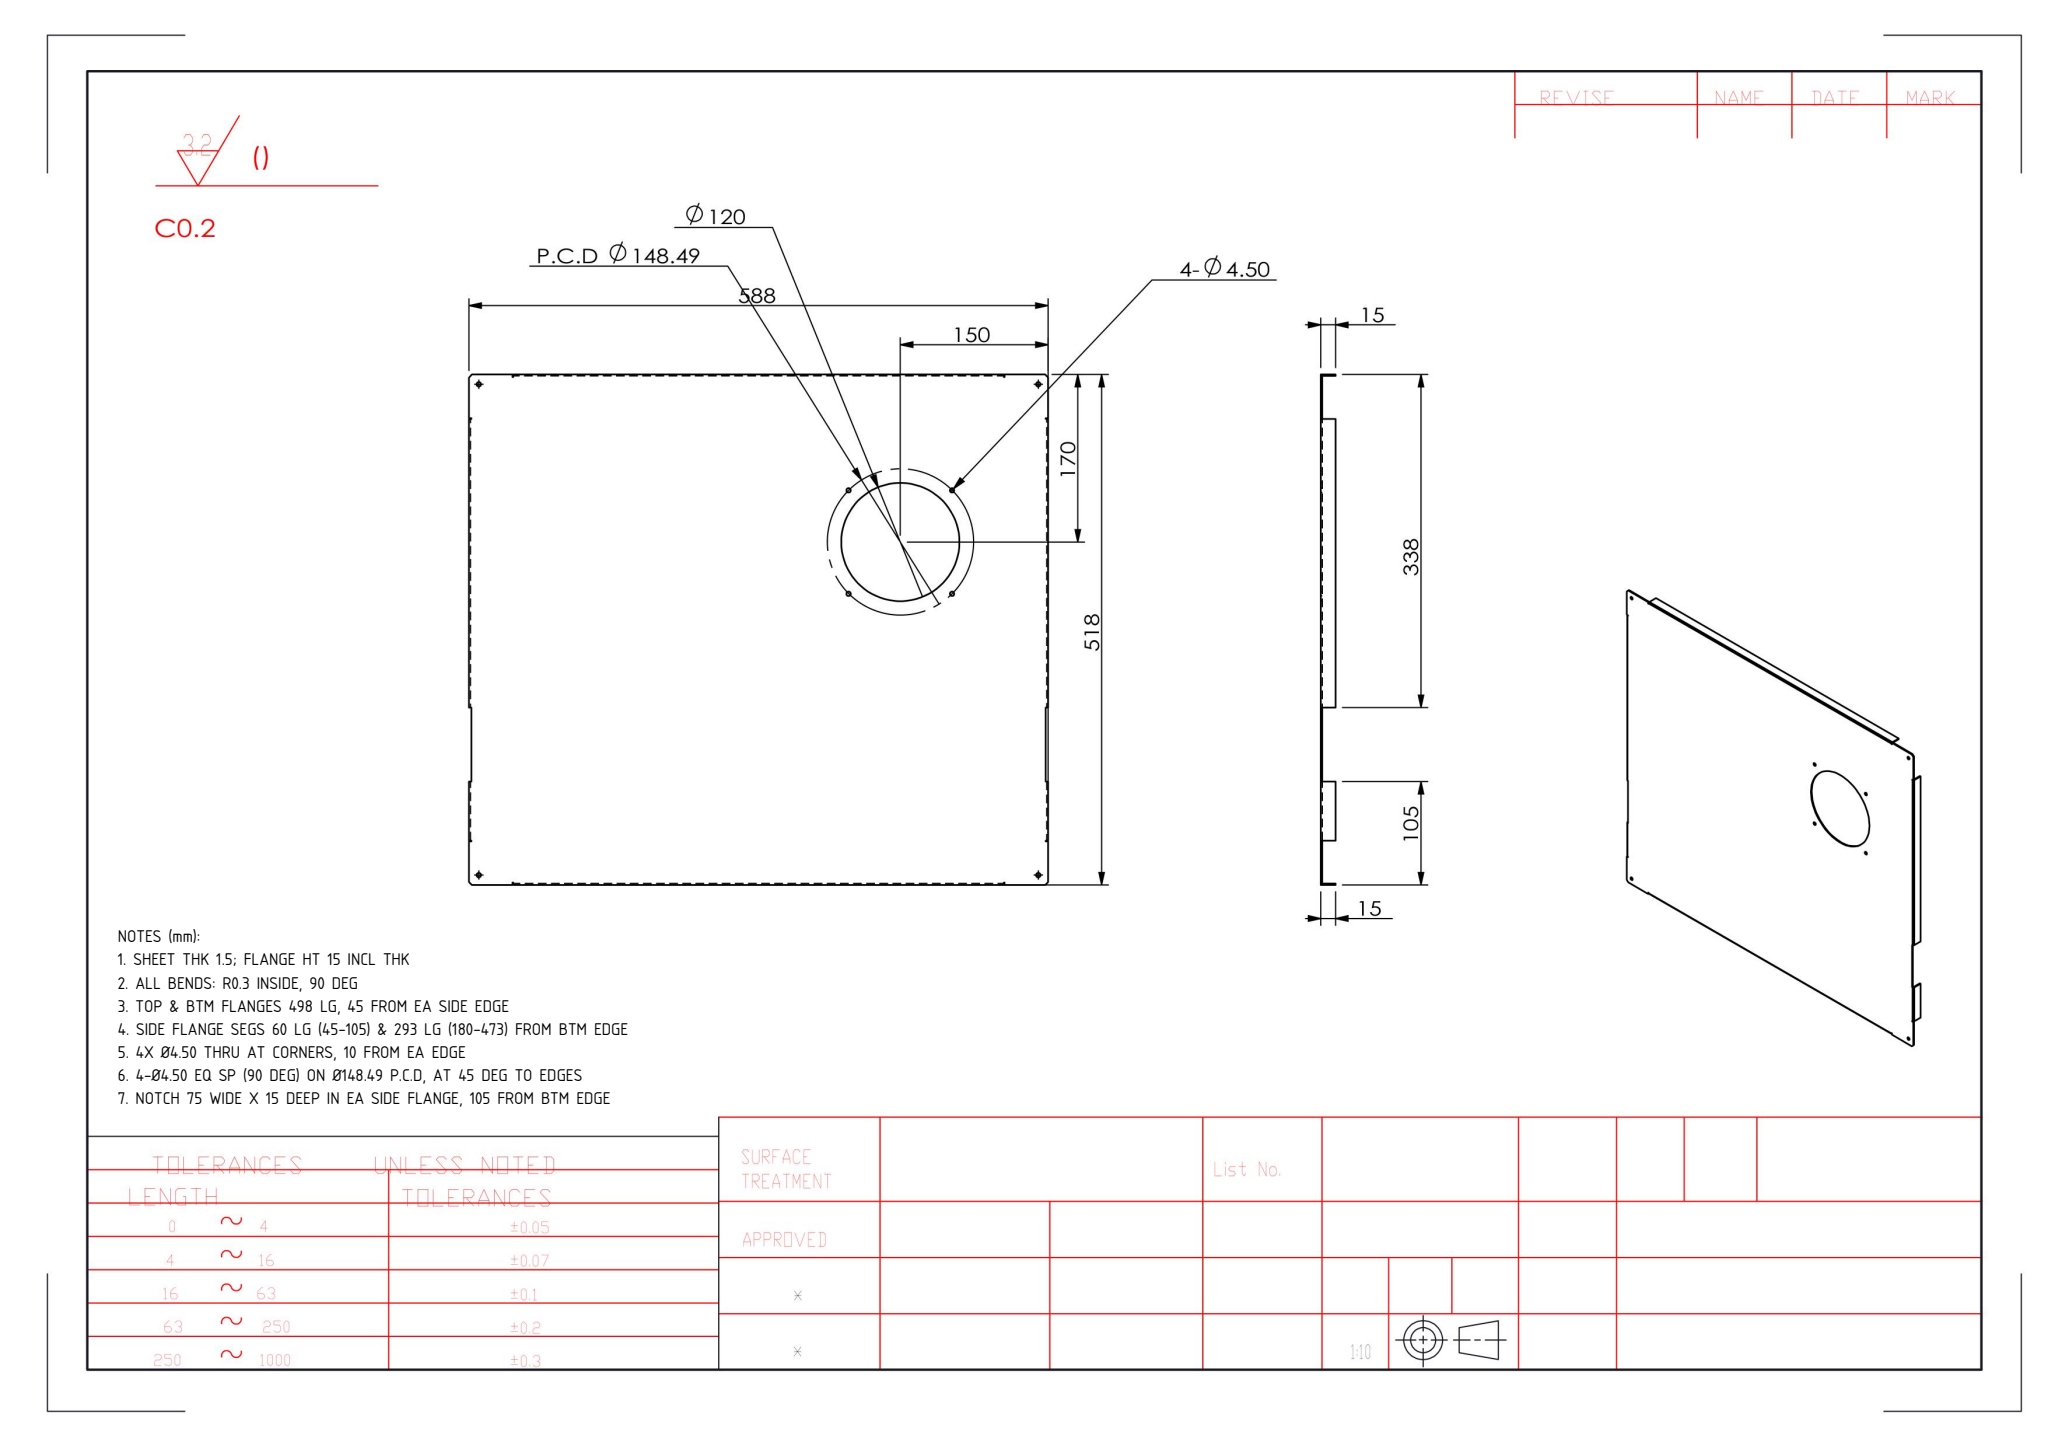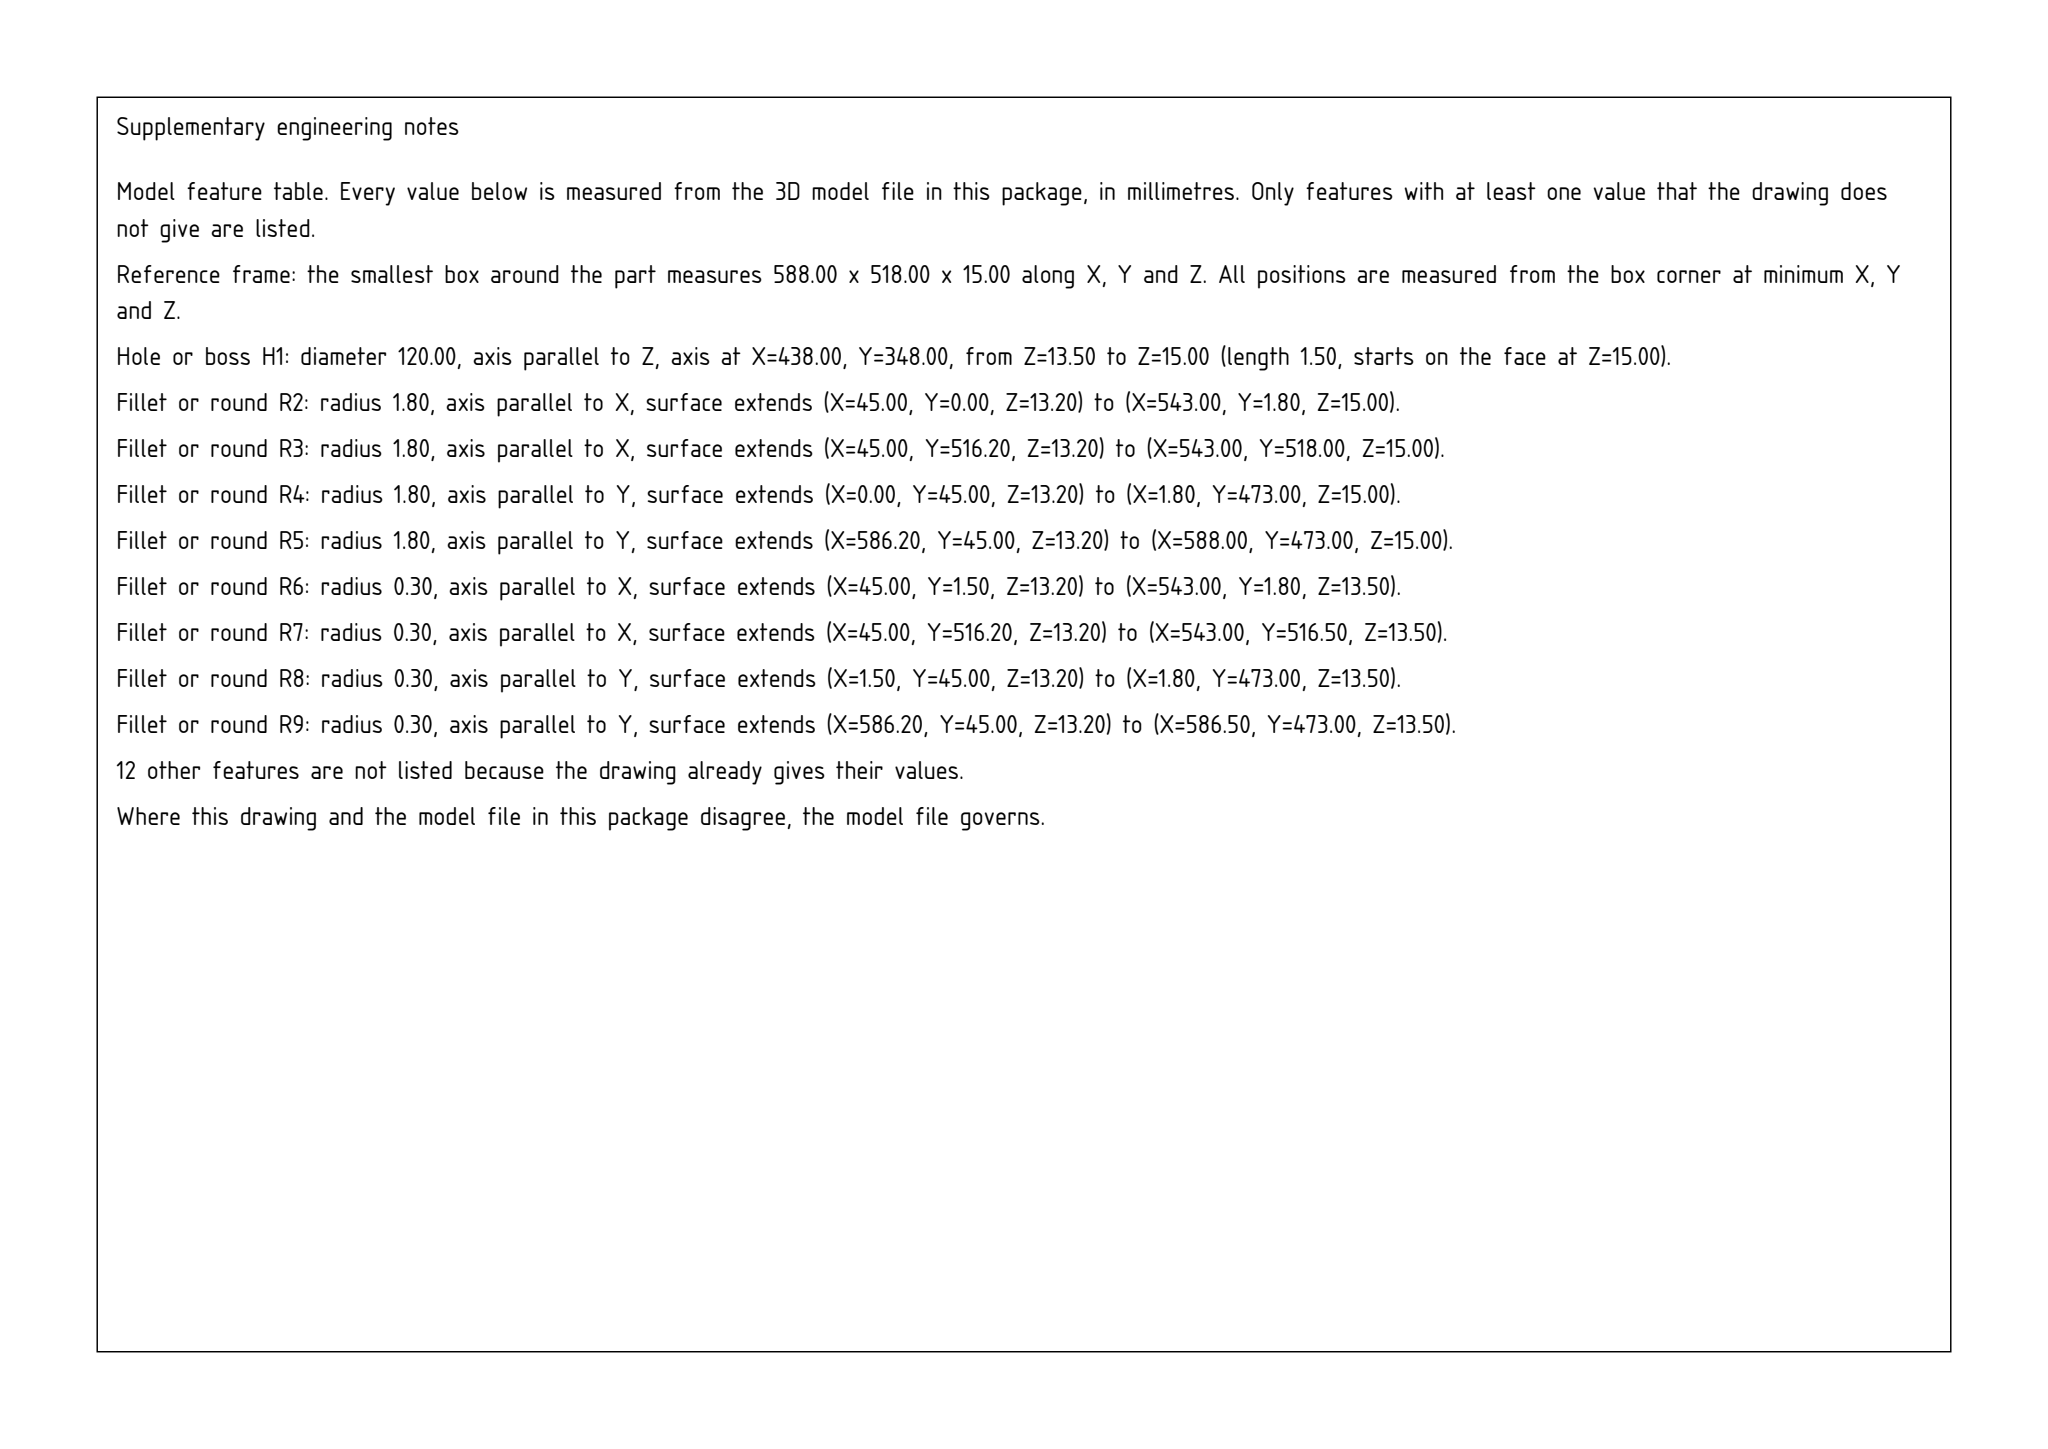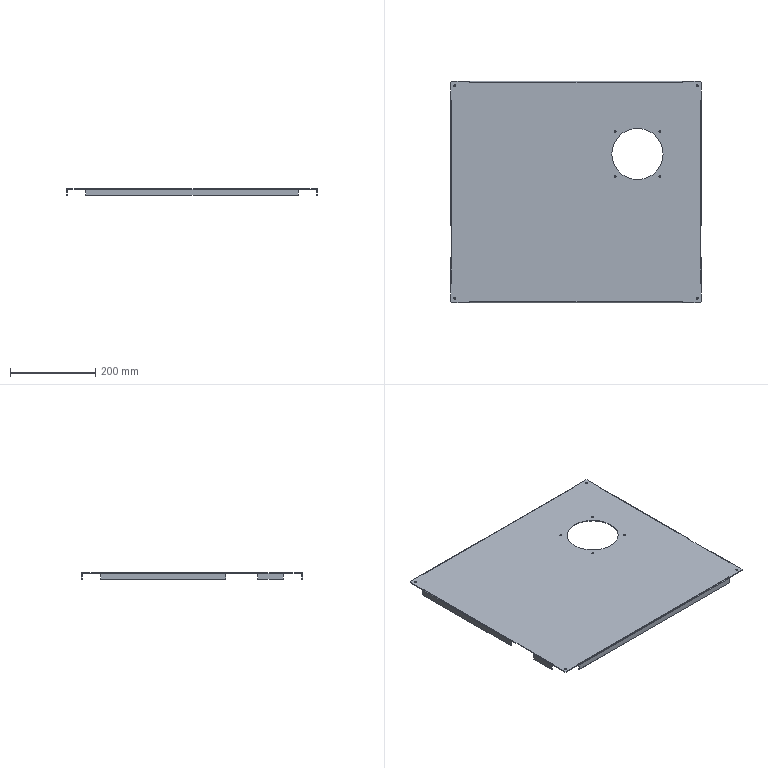Part | SolidWorks | mm | 1 solid | 108 faces | box 588 x 518 x 15 mm | volume 472423 mm3 | plane 78 | cylinder 30 | commonest cylinder face diameters 4.5 x16 3.6 x6 0.6 x6 120 x2
Drawing notes:
SHEET THK 1.5; FLANGE HT 15 INCL THK | from the solid: Hole len 1.5; z planes at 0/13.5/15 => 1.5 sheet, 15 flange
ALL BENDS: R0.3 INSIDE, 90 DEG | from the solid: Bend cyls dia 0.6 (inner R0.3) & 3.6 (outer R1.8) at z=13.2
TOP & BTM FLANGES 498 LG, 45 FROM EA SIDE EDGE | from the solid: x-axis bend cyls len 498 at y=1.8/516.2; x planes 45 & 543
SIDE FLANGE SEGS 60 LG (45-105) & 293 LG (180-473) FROM BTM EDGE | from the solid: y-axis bend cyls len 60 & 293; y planes 45,105,180,473
4X Ø4.50 THRU AT CORNERS, 10 FROM EA EDGE | from the solid: Ø4.5 z-holes at (10,10),(10,508),(578,10),(578,508), len 1.5
4-Ø4.50 EQ SP (90 DEG) ON Ø148.49 P.C.D, AT 45 DEG TO EDGES | from the solid: Ø4.5 holes at 438±52.5, 348±52.5 => R74.245 at 45 deg
NOTCH 75 WIDE X 15 DEEP IN EA SIDE FLANGE, 105 FROM BTM EDGE | from the solid: Gap between side flange segs y=105 to 180; flange ht 15